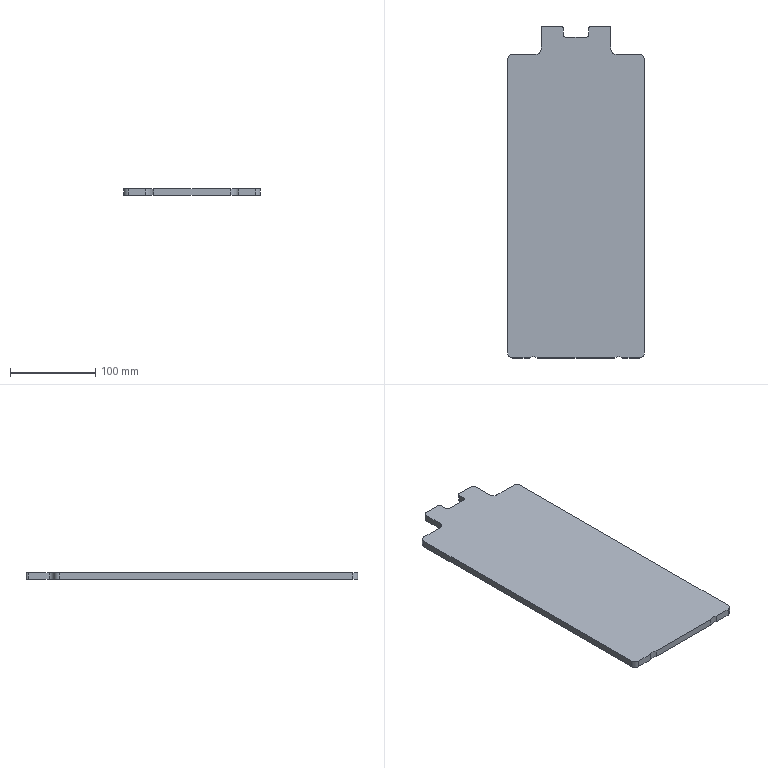CAM job | Mastercam | mm | 6 operations | part box 160 x 389 x 8
1. Contour (Ramp) | 12 - 12 平铣刀
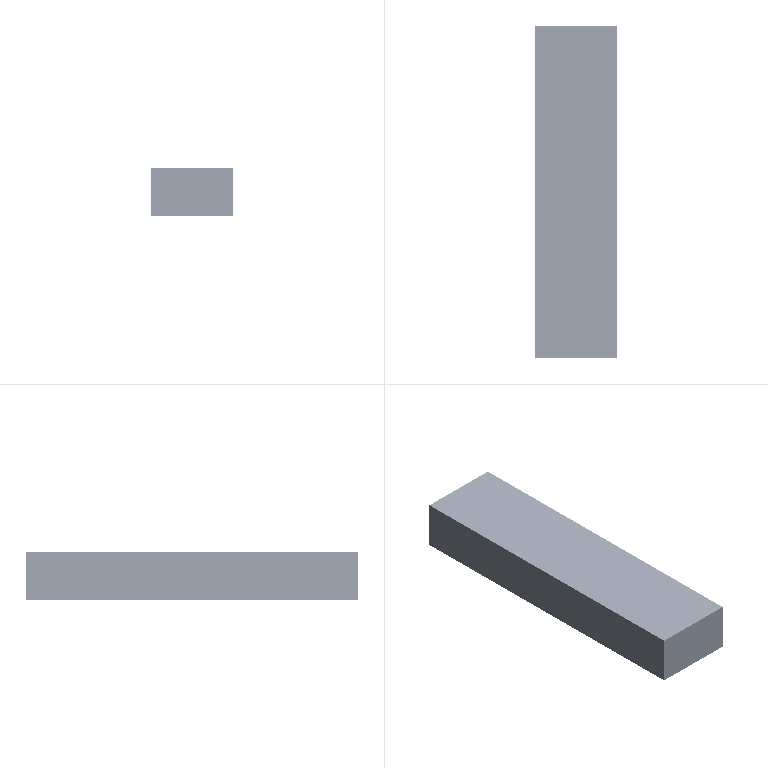2. Contour (Ramp) | 12 - 12 平铣刀
3. Contour (Remachining) | 6 - 6 平铣刀
4. Contour (2D) | 6 - 6 平铣刀
5. Contour (2D chamfer) | 7 - 6 倒角刀
6. Contour (2D chamfer) | 7 - 6 倒角刀